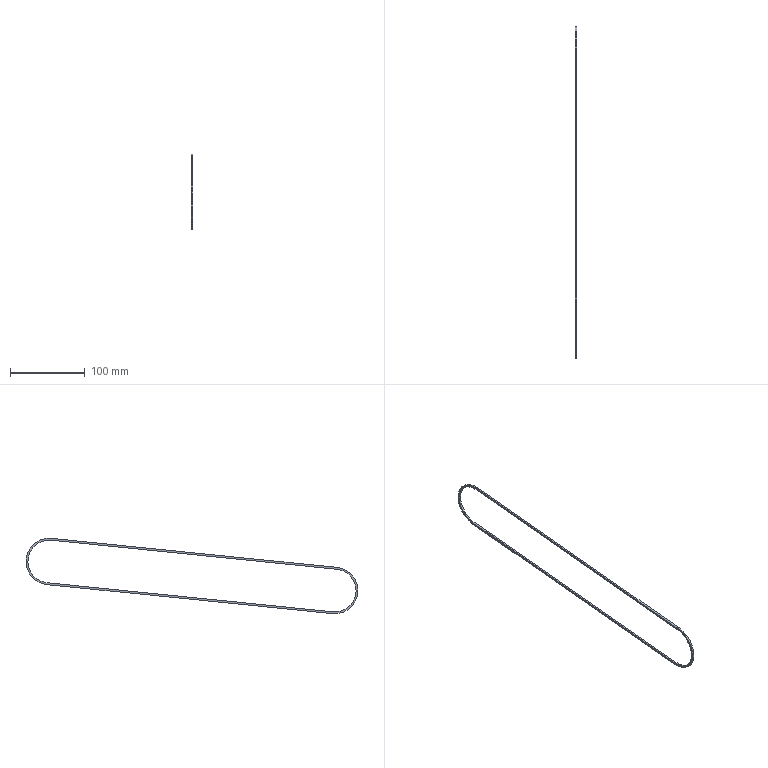Component | SolidWorks | Belt-1 | 1 solid | 12 faces | box 2.2 x 444.2 x 101.04 mm | volume 5255 mm3 | cylinder 6 | plane 6 | commonest cylinder face diameters 57.2 x3 62.2 x3
build123d program:
from build123d import *

# Parameters (mm, degrees)
EXTRUDE_THIN1_DEPTH = 2.2


with BuildPart() as part:
    # Sketch1 → Extrude-Thin1 (new body)
    with BuildSketch(Plane(origin=(0, 0, 0), x_dir=(1, 0, 0), z_dir=(0, 1, 0))):
        with BuildLine():
            Line((-11.523, -194.146), (-50.358, 187.854))
            ThreePointArc((-50.358, 187.854), (-22.563, 221.941), (11.523, 194.146))
            Line((11.523, 194.146), (50.358, -187.854))
            ThreePointArc((50.358, -187.854), (22.563, -221.941), (-11.523, -194.146))
        make_face()
        with BuildLine():
            Line((-9.036, -193.893), (-47.871, 188.107))
            ThreePointArc((-47.871, 188.107), (-22.31, 219.453), (9.036, 193.893))
            Line((9.036, 193.893), (47.871, -188.107))
            ThreePointArc((47.871, -188.107), (22.31, -219.453), (-9.036, -193.893))
        make_face(mode=Mode.SUBTRACT)
    extrude(amount=EXTRUDE_THIN1_DEPTH)


solid = part.part

# Placed as in the assembly
solid = solid.moved(Location((19.145, -156.9, 479.418), (90, 0, -90)))
STEP:
#1=COLOUR_RGB('',0.7922,0.8196,0.9333);
#2=FILL_AREA_STYLE_COLOUR('',#1);
#3=FILL_AREA_STYLE('',(#2));
#4=SURFACE_STYLE_FILL_AREA(#3);
#5=SURFACE_SIDE_STYLE('',(#4));
#6=SURFACE_STYLE_USAGE(.BOTH.,#5);
#7=PRESENTATION_STYLE_ASSIGNMENT((#6));
#8=CARTESIAN_POINT('',(0.7537,1.229,20.759));
#9=VERTEX_POINT('',#8);
#10=CARTESIAN_POINT('',(0.7537,2.445,19.866));
#11=VERTEX_POINT('',#10);
#12=CARTESIAN_POINT('',(0.7537,1.343,19.639));
#13=DIRECTION('',(-1.,0.,0.));
#14=DIRECTION('',(0.,0.9795,0.2012));
#15=AXIS2_PLACEMENT_3D('',#12,#13,#14);
#16=CIRCLE('',#15,1.126);
#17=EDGE_CURVE('',#9,#11,#16,.T.);
#18=ORIENTED_EDGE('',*,*,#17,.T.);
#19=CARTESIAN_POINT('',(0.8404,2.445,19.866));
#20=VERTEX_POINT('',#19);
#21=CARTESIAN_POINT('',(0.7537,2.445,19.866));
#22=DIRECTION('',(1.,-0.,-0.));
#23=VECTOR('',#22,39.37);
#24=LINE('',#21,#23);
#25=EDGE_CURVE('',#11,#20,#24,.T.);
#26=ORIENTED_EDGE('',*,*,#25,.T.);
#27=CARTESIAN_POINT('',(0.8404,1.229,20.759));
#28=VERTEX_POINT('',#27);
#29=CARTESIAN_POINT('',(0.8404,1.343,19.639));
#30=DIRECTION('',(-1.,0.,0.));
#31=DIRECTION('',(0.,0.9795,0.2012));
#32=AXIS2_PLACEMENT_3D('',#29,#30,#31);
#33=CIRCLE('',#32,1.126);
#34=EDGE_CURVE('',#28,#20,#33,.T.);
#35=ORIENTED_EDGE('',*,*,#34,.F.);
#36=CARTESIAN_POINT('',(0.7537,1.229,20.759));
#37=DIRECTION('',(1.,-0.,-0.));
#38=VECTOR('',#37,39.37);
#39=LINE('',#36,#38);
#40=EDGE_CURVE('',#9,#28,#39,.T.);
#41=ORIENTED_EDGE('',*,*,#40,.F.);
#42=EDGE_LOOP('',(#18,#26,#35,#41));
#43=FACE_OUTER_BOUND('',#42,.T.);
#44=CARTESIAN_POINT('',(0.7537,1.343,19.639));
#45=DIRECTION('',(1.,-0.,-0.));
#46=DIRECTION('',(0.,0.9795,0.2012));
#47=AXIS2_PLACEMENT_3D('',#44,#45,#46);
#48=CYLINDRICAL_SURFACE('',#47,1.126);
#49=ADVANCED_FACE('',(#43),#48,.F.);
#50=CARTESIAN_POINT('',(0.7537,2.542,19.886));
#51=VERTEX_POINT('',#50);
#52=CARTESIAN_POINT('',(0.7537,1.466,18.421));
#53=VERTEX_POINT('',#52);
#54=CARTESIAN_POINT('',(0.7537,1.343,19.639));
#55=DIRECTION('',(-1.,0.,0.));
#56=DIRECTION('',(-0.,0.2012,-0.9795));
#57=AXIS2_PLACEMENT_3D('',#54,#55,#56);
#58=CIRCLE('',#57,1.224);
#59=EDGE_CURVE('',#51,#53,#58,.T.);
#60=ORIENTED_EDGE('',*,*,#59,.F.);
#61=CARTESIAN_POINT('',(0.8404,2.542,19.886));
#62=VERTEX_POINT('',#61);
#63=CARTESIAN_POINT('',(0.7537,2.542,19.886));
#64=DIRECTION('',(1.,-0.,-0.));
#65=VECTOR('',#64,39.37);
#66=LINE('',#63,#65);
#67=EDGE_CURVE('',#51,#62,#66,.T.);
#68=ORIENTED_EDGE('',*,*,#67,.T.);
#69=CARTESIAN_POINT('',(0.8404,1.466,18.421));
#70=VERTEX_POINT('',#69);
#71=CARTESIAN_POINT('',(0.8404,1.343,19.639));
#72=DIRECTION('',(-1.,0.,0.));
#73=DIRECTION('',(-0.,0.2012,-0.9795));
#74=AXIS2_PLACEMENT_3D('',#71,#72,#73);
#75=CIRCLE('',#74,1.224);
#76=EDGE_CURVE('',#62,#70,#75,.T.);
#77=ORIENTED_EDGE('',*,*,#76,.T.);
#78=CARTESIAN_POINT('',(0.7537,1.466,18.421));
#79=DIRECTION('',(1.,-0.,-0.));
#80=VECTOR('',#79,39.37);
#81=LINE('',#78,#80);
#82=EDGE_CURVE('',#53,#70,#81,.T.);
#83=ORIENTED_EDGE('',*,*,#82,.F.);
#84=EDGE_LOOP('',(#60,#68,#77,#83));
#85=FACE_OUTER_BOUND('',#84,.T.);
#86=CARTESIAN_POINT('',(0.7537,1.343,19.639));
#87=DIRECTION('',(1.,-0.,-0.));
#88=DIRECTION('',(0.,0.9795,0.2012));
#89=AXIS2_PLACEMENT_3D('',#86,#87,#88);
#90=CYLINDRICAL_SURFACE('',#89,1.224);
#91=ADVANCED_FACE('',(#85),#90,.T.);
#92=CARTESIAN_POINT('',(0.7537,1.219,20.857));
#93=VERTEX_POINT('',#92);
#94=CARTESIAN_POINT('',(0.7537,1.343,19.639));
#95=DIRECTION('',(-1.,0.,0.));
#96=DIRECTION('',(-0.,0.2012,-0.9795));
#97=AXIS2_PLACEMENT_3D('',#94,#95,#96);
#98=CIRCLE('',#97,1.224);
#99=EDGE_CURVE('',#93,#51,#98,.T.);
#100=ORIENTED_EDGE('',*,*,#99,.T.);
#101=ORIENTED_EDGE('',*,*,#59,.T.);
#102=CARTESIAN_POINT('',(0.7537,-13.573,16.892));
#103=VERTEX_POINT('',#102);
#104=CARTESIAN_POINT('',(0.7537,1.466,18.421));
#105=DIRECTION('',(-0.,-0.9949,-0.1011));
#106=VECTOR('',#105,39.37);
#107=LINE('',#104,#106);
#108=EDGE_CURVE('',#53,#103,#107,.T.);
#109=ORIENTED_EDGE('',*,*,#108,.T.);
#110=CARTESIAN_POINT('',(0.7537,-13.821,19.328));
#111=VERTEX_POINT('',#110);
#112=CARTESIAN_POINT('',(0.7537,-13.697,18.11));
#113=DIRECTION('',(-1.,0.,0.));
#114=DIRECTION('',(-0.,0.2012,-0.9795));
#115=AXIS2_PLACEMENT_3D('',#112,#113,#114);
#116=CIRCLE('',#115,1.224);
#117=EDGE_CURVE('',#103,#111,#116,.T.);
#118=ORIENTED_EDGE('',*,*,#117,.T.);
#119=CARTESIAN_POINT('',(0.7537,1.219,20.857));
#120=DIRECTION('',(0.,0.9949,0.1011));
#121=VECTOR('',#120,39.37);
#122=LINE('',#119,#121);
#123=EDGE_CURVE('',#111,#93,#122,.T.);
#124=ORIENTED_EDGE('',*,*,#123,.T.);
#125=EDGE_LOOP('',(#100,#101,#109,#118,#124));
#126=FACE_OUTER_BOUND('',#125,.T.);
#127=ORIENTED_EDGE('',*,*,#17,.F.);
#128=CARTESIAN_POINT('',(0.7537,-13.811,19.23));
#129=VERTEX_POINT('',#128);
#130=CARTESIAN_POINT('',(0.7537,1.229,20.759));
#131=DIRECTION('',(0.,0.9949,0.1011));
#132=VECTOR('',#131,39.37);
#133=LINE('',#130,#132);
#134=EDGE_CURVE('',#129,#9,#133,.T.);
#135=ORIENTED_EDGE('',*,*,#134,.F.);
#136=CARTESIAN_POINT('',(0.7537,-13.583,16.99));
#137=VERTEX_POINT('',#136);
#138=CARTESIAN_POINT('',(0.7537,-13.697,18.11));
#139=DIRECTION('',(-1.,0.,0.));
#140=DIRECTION('',(0.,0.9795,0.2012));
#141=AXIS2_PLACEMENT_3D('',#138,#139,#140);
#142=CIRCLE('',#141,1.126);
#143=EDGE_CURVE('',#137,#129,#142,.T.);
#144=ORIENTED_EDGE('',*,*,#143,.F.);
#145=CARTESIAN_POINT('',(0.7537,1.456,18.519));
#146=VERTEX_POINT('',#145);
#147=CARTESIAN_POINT('',(0.7537,-13.583,16.99));
#148=DIRECTION('',(-0.,-0.9949,-0.1011));
#149=VECTOR('',#148,39.37);
#150=LINE('',#147,#149);
#151=EDGE_CURVE('',#146,#137,#150,.T.);
#152=ORIENTED_EDGE('',*,*,#151,.F.);
#153=CARTESIAN_POINT('',(0.7537,1.343,19.639));
#154=DIRECTION('',(-1.,0.,0.));
#155=DIRECTION('',(0.,0.9795,0.2012));
#156=AXIS2_PLACEMENT_3D('',#153,#154,#155);
#157=CIRCLE('',#156,1.126);
#158=EDGE_CURVE('',#11,#146,#157,.T.);
#159=ORIENTED_EDGE('',*,*,#158,.F.);
#160=EDGE_LOOP('',(#127,#135,#144,#152,#159));
#161=FACE_BOUND('',#160,.T.);
#162=CARTESIAN_POINT('',(0.7537,1.343,19.639));
#163=DIRECTION('',(1.,-0.,-0.));
#164=DIRECTION('',(0.,0.9795,0.2012));
#165=AXIS2_PLACEMENT_3D('',#162,#163,#164);
#166=PLANE('',#165);
#167=ADVANCED_FACE('',(#126,#161),#166,.F.);
#168=CARTESIAN_POINT('',(0.8404,1.219,20.857));
#169=VERTEX_POINT('',#168);
#170=CARTESIAN_POINT('',(0.8404,1.343,19.639));
#171=DIRECTION('',(-1.,0.,0.));
#172=DIRECTION('',(-0.,0.2012,-0.9795));
#173=AXIS2_PLACEMENT_3D('',#170,#171,#172);
#174=CIRCLE('',#173,1.224);
#175=EDGE_CURVE('',#169,#62,#174,.T.);
#176=ORIENTED_EDGE('',*,*,#175,.F.);
#177=CARTESIAN_POINT('',(0.8404,-13.821,19.328));
#178=VERTEX_POINT('',#177);
#179=CARTESIAN_POINT('',(0.8404,1.219,20.857));
#180=DIRECTION('',(0.,0.9949,0.1011));
#181=VECTOR('',#180,39.37);
#182=LINE('',#179,#181);
#183=EDGE_CURVE('',#178,#169,#182,.T.);
#184=ORIENTED_EDGE('',*,*,#183,.F.);
#185=CARTESIAN_POINT('',(0.8404,-13.573,16.892));
#186=VERTEX_POINT('',#185);
#187=CARTESIAN_POINT('',(0.8404,-13.697,18.11));
#188=DIRECTION('',(-1.,0.,0.));
#189=DIRECTION('',(-0.,0.2012,-0.9795));
#190=AXIS2_PLACEMENT_3D('',#187,#188,#189);
#191=CIRCLE('',#190,1.224);
#192=EDGE_CURVE('',#186,#178,#191,.T.);
#193=ORIENTED_EDGE('',*,*,#192,.F.);
#194=CARTESIAN_POINT('',(0.8404,1.466,18.421));
#195=DIRECTION('',(-0.,-0.9949,-0.1011));
#196=VECTOR('',#195,39.37);
#197=LINE('',#194,#196);
#198=EDGE_CURVE('',#70,#186,#197,.T.);
#199=ORIENTED_EDGE('',*,*,#198,.F.);
#200=ORIENTED_EDGE('',*,*,#76,.F.);
#201=EDGE_LOOP('',(#176,#184,#193,#199,#200));
#202=FACE_OUTER_BOUND('',#201,.T.);
#203=CARTESIAN_POINT('',(0.8404,-13.811,19.23));
#204=VERTEX_POINT('',#203);
#205=CARTESIAN_POINT('',(0.8404,1.229,20.759));
#206=DIRECTION('',(0.,0.9949,0.1011));
#207=VECTOR('',#206,39.37);
#208=LINE('',#205,#207);
#209=EDGE_CURVE('',#204,#28,#208,.T.);
#210=ORIENTED_EDGE('',*,*,#209,.T.);
#211=ORIENTED_EDGE('',*,*,#34,.T.);
#212=CARTESIAN_POINT('',(0.8404,1.456,18.519));
#213=VERTEX_POINT('',#212);
#214=CARTESIAN_POINT('',(0.8404,1.343,19.639));
#215=DIRECTION('',(-1.,0.,0.));
#216=DIRECTION('',(0.,0.9795,0.2012));
#217=AXIS2_PLACEMENT_3D('',#214,#215,#216);
#218=CIRCLE('',#217,1.126);
#219=EDGE_CURVE('',#20,#213,#218,.T.);
#220=ORIENTED_EDGE('',*,*,#219,.T.);
#221=CARTESIAN_POINT('',(0.8404,-13.583,16.99));
#222=VERTEX_POINT('',#221);
#223=CARTESIAN_POINT('',(0.8404,-13.583,16.99));
#224=DIRECTION('',(-0.,-0.9949,-0.1011));
#225=VECTOR('',#224,39.37);
#226=LINE('',#223,#225);
#227=EDGE_CURVE('',#213,#222,#226,.T.);
#228=ORIENTED_EDGE('',*,*,#227,.T.);
#229=CARTESIAN_POINT('',(0.8404,-13.697,18.11));
#230=DIRECTION('',(-1.,0.,0.));
#231=DIRECTION('',(0.,0.9795,0.2012));
#232=AXIS2_PLACEMENT_3D('',#229,#230,#231);
#233=CIRCLE('',#232,1.126);
#234=EDGE_CURVE('',#222,#204,#233,.T.);
#235=ORIENTED_EDGE('',*,*,#234,.T.);
#236=EDGE_LOOP('',(#210,#211,#220,#228,#235));
#237=FACE_BOUND('',#236,.T.);
#238=CARTESIAN_POINT('',(0.8404,1.343,19.639));
#239=DIRECTION('',(1.,-0.,-0.));
#240=DIRECTION('',(0.,0.9795,0.2012));
#241=AXIS2_PLACEMENT_3D('',#238,#239,#240);
#242=PLANE('',#241);
#243=ADVANCED_FACE('',(#202,#237),#242,.T.);
#244=ORIENTED_EDGE('',*,*,#67,.F.);
#245=ORIENTED_EDGE('',*,*,#99,.F.);
#246=CARTESIAN_POINT('',(0.7537,1.219,20.857));
#247=DIRECTION('',(1.,-0.,-0.));
#248=VECTOR('',#247,39.37);
#249=LINE('',#246,#248);
#250=EDGE_CURVE('',#93,#169,#249,.T.);
#251=ORIENTED_EDGE('',*,*,#250,.T.);
#252=ORIENTED_EDGE('',*,*,#175,.T.);
#253=EDGE_LOOP('',(#244,#245,#251,#252));
#254=FACE_OUTER_BOUND('',#253,.T.);
#255=CARTESIAN_POINT('',(0.7537,1.343,19.639));
#256=DIRECTION('',(1.,-0.,-0.));
#257=DIRECTION('',(0.,0.9795,0.2012));
#258=AXIS2_PLACEMENT_3D('',#255,#256,#257);
#259=CYLINDRICAL_SURFACE('',#258,1.224);
#260=ADVANCED_FACE('',(#254),#259,.T.);
#261=ORIENTED_EDGE('',*,*,#198,.T.);
#262=CARTESIAN_POINT('',(0.7537,-13.573,16.892));
#263=DIRECTION('',(1.,-0.,-0.));
#264=VECTOR('',#263,39.37);
#265=LINE('',#262,#264);
#266=EDGE_CURVE('',#103,#186,#265,.T.);
#267=ORIENTED_EDGE('',*,*,#266,.F.);
#268=ORIENTED_EDGE('',*,*,#108,.F.);
#269=ORIENTED_EDGE('',*,*,#82,.T.);
#270=EDGE_LOOP('',(#261,#267,#268,#269));
#271=FACE_OUTER_BOUND('',#270,.T.);
#272=CARTESIAN_POINT('',(0.7537,1.466,18.421));
#273=DIRECTION('',(0.,-0.1011,0.9949));
#274=DIRECTION('',(0.,0.9949,0.1011));
#275=AXIS2_PLACEMENT_3D('',#272,#273,#274);
#276=PLANE('',#275);
#277=ADVANCED_FACE('',(#271),#276,.F.);
#278=ORIENTED_EDGE('',*,*,#192,.T.);
#279=CARTESIAN_POINT('',(0.7537,-13.821,19.328));
#280=DIRECTION('',(1.,-0.,-0.));
#281=VECTOR('',#280,39.37);
#282=LINE('',#279,#281);
#283=EDGE_CURVE('',#111,#178,#282,.T.);
#284=ORIENTED_EDGE('',*,*,#283,.F.);
#285=ORIENTED_EDGE('',*,*,#117,.F.);
#286=ORIENTED_EDGE('',*,*,#266,.T.);
#287=EDGE_LOOP('',(#278,#284,#285,#286));
#288=FACE_OUTER_BOUND('',#287,.T.);
#289=CARTESIAN_POINT('',(0.7537,-13.697,18.11));
#290=DIRECTION('',(1.,-0.,-0.));
#291=DIRECTION('',(0.,0.9795,0.2012));
#292=AXIS2_PLACEMENT_3D('',#289,#290,#291);
#293=CYLINDRICAL_SURFACE('',#292,1.224);
#294=ADVANCED_FACE('',(#288),#293,.T.);
#295=ORIENTED_EDGE('',*,*,#183,.T.);
#296=ORIENTED_EDGE('',*,*,#250,.F.);
#297=ORIENTED_EDGE('',*,*,#123,.F.);
#298=ORIENTED_EDGE('',*,*,#283,.T.);
#299=EDGE_LOOP('',(#295,#296,#297,#298));
#300=FACE_OUTER_BOUND('',#299,.T.);
#301=CARTESIAN_POINT('',(0.7537,1.219,20.857));
#302=DIRECTION('',(-0.,0.1011,-0.9949));
#303=DIRECTION('',(-0.,-0.9949,-0.1011));
#304=AXIS2_PLACEMENT_3D('',#301,#302,#303);
#305=PLANE('',#304);
#306=ADVANCED_FACE('',(#300),#305,.F.);
#307=ORIENTED_EDGE('',*,*,#25,.F.);
#308=ORIENTED_EDGE('',*,*,#158,.T.);
#309=CARTESIAN_POINT('',(0.7537,1.456,18.519));
#310=DIRECTION('',(1.,-0.,-0.));
#311=VECTOR('',#310,39.37);
#312=LINE('',#309,#311);
#313=EDGE_CURVE('',#146,#213,#312,.T.);
#314=ORIENTED_EDGE('',*,*,#313,.T.);
#315=ORIENTED_EDGE('',*,*,#219,.F.);
#316=EDGE_LOOP('',(#307,#308,#314,#315));
#317=FACE_OUTER_BOUND('',#316,.T.);
#318=CARTESIAN_POINT('',(0.7537,1.343,19.639));
#319=DIRECTION('',(1.,-0.,-0.));
#320=DIRECTION('',(0.,0.9795,0.2012));
#321=AXIS2_PLACEMENT_3D('',#318,#319,#320);
#322=CYLINDRICAL_SURFACE('',#321,1.126);
#323=ADVANCED_FACE('',(#317),#322,.F.);
#324=ORIENTED_EDGE('',*,*,#227,.F.);
#325=ORIENTED_EDGE('',*,*,#313,.F.);
#326=ORIENTED_EDGE('',*,*,#151,.T.);
#327=CARTESIAN_POINT('',(0.7537,-13.583,16.99));
#328=DIRECTION('',(1.,-0.,-0.));
#329=VECTOR('',#328,39.37);
#330=LINE('',#327,#329);
#331=EDGE_CURVE('',#137,#222,#330,.T.);
#332=ORIENTED_EDGE('',*,*,#331,.T.);
#333=EDGE_LOOP('',(#324,#325,#326,#332));
#334=FACE_OUTER_BOUND('',#333,.T.);
#335=CARTESIAN_POINT('',(0.7537,-13.583,16.99));
#336=DIRECTION('',(0.,-0.1011,0.9949));
#337=DIRECTION('',(0.,0.9949,0.1011));
#338=AXIS2_PLACEMENT_3D('',#335,#336,#337);
#339=PLANE('',#338);
#340=ADVANCED_FACE('',(#334),#339,.T.);
#341=ORIENTED_EDGE('',*,*,#234,.F.);
#342=ORIENTED_EDGE('',*,*,#331,.F.);
#343=ORIENTED_EDGE('',*,*,#143,.T.);
#344=CARTESIAN_POINT('',(0.7537,-13.811,19.23));
#345=DIRECTION('',(1.,-0.,-0.));
#346=VECTOR('',#345,39.37);
#347=LINE('',#344,#346);
#348=EDGE_CURVE('',#129,#204,#347,.T.);
#349=ORIENTED_EDGE('',*,*,#348,.T.);
#350=EDGE_LOOP('',(#341,#342,#343,#349));
#351=FACE_OUTER_BOUND('',#350,.T.);
#352=CARTESIAN_POINT('',(0.7537,-13.697,18.11));
#353=DIRECTION('',(1.,-0.,-0.));
#354=DIRECTION('',(0.,0.9795,0.2012));
#355=AXIS2_PLACEMENT_3D('',#352,#353,#354);
#356=CYLINDRICAL_SURFACE('',#355,1.126);
#357=ADVANCED_FACE('',(#351),#356,.F.);
#358=ORIENTED_EDGE('',*,*,#209,.F.);
#359=ORIENTED_EDGE('',*,*,#348,.F.);
#360=ORIENTED_EDGE('',*,*,#134,.T.);
#361=ORIENTED_EDGE('',*,*,#40,.T.);
#362=EDGE_LOOP('',(#358,#359,#360,#361));
#363=FACE_OUTER_BOUND('',#362,.T.);
#364=CARTESIAN_POINT('',(0.7537,1.229,20.759));
#365=DIRECTION('',(-0.,0.1011,-0.9949));
#366=DIRECTION('',(-0.,-0.9949,-0.1011));
#367=AXIS2_PLACEMENT_3D('',#364,#365,#366);
#368=PLANE('',#367);
#369=ADVANCED_FACE('',(#363),#368,.T.);
#370=CLOSED_SHELL('',(#49,#91,#167,#243,#260,#277,#294,#306,#323,#340,#357,#369));
#371=MANIFOLD_SOLID_BREP('',#370);
#372=STYLED_ITEM('',(#7),#371);
#373=PRESENTATION_LAYER_ASSIGNMENT('','',(#372));
#374=CARTESIAN_POINT('',(0.,0.,0.));
#375=DIRECTION('',(0.,0.,1.));
#376=DIRECTION('',(1.,0.,0.));
#377=AXIS2_PLACEMENT_3D('',#374,#375,#376);
#378=(LENGTH_UNIT()NAMED_UNIT(*)SI_UNIT($,.METRE.));
#379=LENGTH_MEASURE_WITH_UNIT(LENGTH_MEASURE(0.0254),#378);
#380=DIMENSIONAL_EXPONENTS(1.,0.,0.,0.,0.,0.,0.);
#381=(CONVERSION_BASED_UNIT('',#379)LENGTH_UNIT()NAMED_UNIT(#380));
#382=UNCERTAINTY_MEASURE_WITH_UNIT(LENGTH_MEASURE(0.00001),#381,'','');
#383=(NAMED_UNIT(*)PLANE_ANGLE_UNIT()SI_UNIT($,.RADIAN.));
#384=(NAMED_UNIT(*)SI_UNIT($,.STERADIAN.)SOLID_ANGLE_UNIT());
#385=(GEOMETRIC_REPRESENTATION_CONTEXT(3)GLOBAL_UNCERTAINTY_ASSIGNED_CONTEXT((#382))GLOBAL_UNIT_ASSIGNED_CONTEXT((#381,#383,#384))REPRESENTATION_CONTEXT('',''));
#386=ADVANCED_BREP_SHAPE_REPRESENTATION('',(#371,#377),#385);
#387=(LENGTH_UNIT()NAMED_UNIT(*)SI_UNIT($,.METRE.));
#388=LENGTH_MEASURE_WITH_UNIT(LENGTH_MEASURE(0.0254),#387);
#389=DIMENSIONAL_EXPONENTS(1.,0.,0.,0.,0.,0.,0.);
#390=(CONVERSION_BASED_UNIT('',#388)LENGTH_UNIT()NAMED_UNIT(#389));
#391=UNCERTAINTY_MEASURE_WITH_UNIT(LENGTH_MEASURE(0.00001),#390,'','');
#392=(NAMED_UNIT(*)PLANE_ANGLE_UNIT()SI_UNIT($,.RADIAN.));
#393=(NAMED_UNIT(*)SI_UNIT($,.STERADIAN.)SOLID_ANGLE_UNIT());
#394=(GEOMETRIC_REPRESENTATION_CONTEXT(3)GLOBAL_UNCERTAINTY_ASSIGNED_CONTEXT((#391))GLOBAL_UNIT_ASSIGNED_CONTEXT((#390,#392,#393))REPRESENTATION_CONTEXT('',''));
#395=MECHANICAL_DESIGN_GEOMETRIC_PRESENTATION_REPRESENTATION('',(#372),#394);